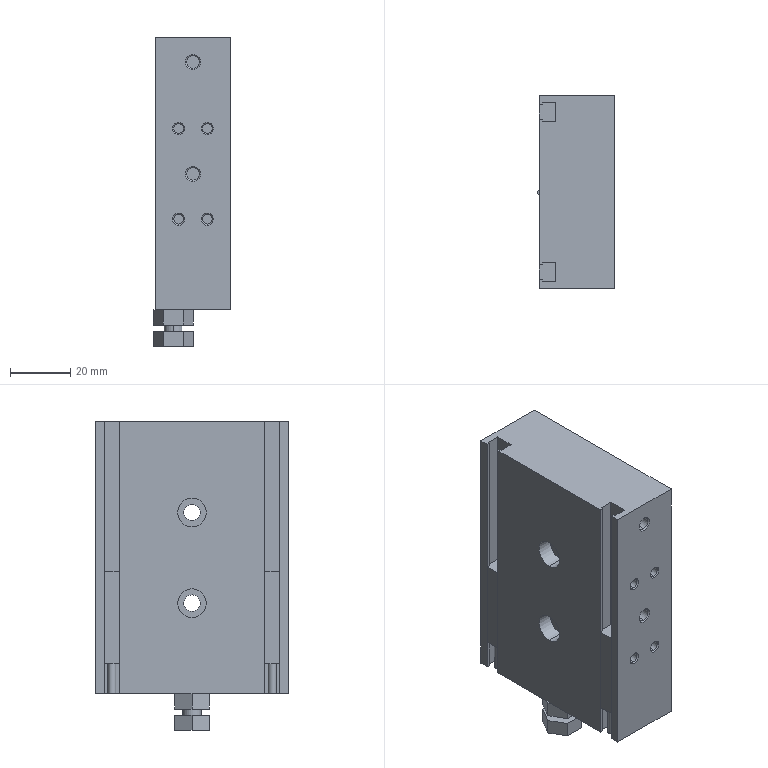Component | SolidWorks | P-SLJ-005-3_CXSM20-20-Z73-1_body CXSM20-20-Z73-1 | 1 solid | 147 faces | box 25.64 x 64 x 102 mm | volume 135415 mm3 | plane 75 | cylinder 44 | cone 28 | commonest cylinder face diameters 3.24 x16 4.13 x8 10.2 x4 2.7 x4 9.5 x4 5.5 x4 6 x4
build123d program:
from build123d import *

# Parameters (mm, degrees)
EXTRUDE1_DEPTH = 90
SKETCH2_W      = 12
SKETCH2_H      = 3
EXTRUDE2_DEPTH = 5
EXTRUDE3_DEPTH = 5
EXTRUDE4_DEPTH = 30.5
EXTRUDE5_DEPTH = 30.5
SKETCH9_R      = 1.35
EXTRUDE6_DEPTH = 10
SKETCH10_R     = 1.35
EXTRUDE7_DEPTH = 10
SKETCH23_R     = 5.1
EXTRUDE8_DEPTH = 22
SKETCH24_R     = 5.1
EXTRUDE9_DEPTH = 22


with BuildPart() as part:
    # Sketch1 → Extrude1 (new body)
    with BuildSketch(Plane.XY):
        Polygon((-32, 0), (32, 0), (32, 25), (29, 25), (29, 24), (29.65, 24), (29.65, 19.5), (23.35, 19.5), (23.35, 24), (24, 24), (24, 25), (-24, 25), (-24, 24), (-23.35, 24), (-23.35, 19.5), (-29.65, 19.5), (-29.65, 24), (-29, 24), (-29, 25), (-32, 25), align=None)
    extrude(amount=-EXTRUDE1_DEPTH)

    # Sketch2 → Revolve1 (revolve)
    with BuildSketch(Plane(origin=(0, 0, 0), x_dir=(0, 0, -1), z_dir=(1, 0, 0)), mode=Mode.PRIVATE) as revolve1_sk:
        with Locations((-6, 20.5)):
            Rectangle(SKETCH2_W, SKETCH2_H)
    revolve(revolve1_sk.sketch.rotate(Axis((0, 19, 0), (0, 0, 1)), 270), axis=Axis((0, 19, 0), (0, 0, 1)))

    # Sketch3 → Extrude2 (add)
    with BuildSketch(Plane.XY):
        Polygon((-5.75, 22.32), (-5.75, 15.68), (0, 12.36), (5.75, 15.68), (5.75, 22.32), (0, 25.64), align=None)
    extrude(amount=EXTRUDE2_DEPTH)

    # Sketch4 → Extrude3 (add)
    with BuildSketch(Plane.XY.offset(11.99)):
        Polygon((-5.75, 22.32), (-5.75, 15.68), (0, 12.36), (5.75, 15.68), (5.75, 22.32), (0, 25.64), align=None)
    extrude(amount=-EXTRUDE3_DEPTH)

    # Sketch5 → Cut-Revolve1 (revolve, cut)
    with BuildSketch(Plane(origin=(0, 0, 0), x_dir=(0, 0, -1), z_dir=(1, 0, 0)), mode=Mode.PRIVATE) as cut_revolve1_sk:
        Polygon((30, -0.5), (26.5, -0.5), (27.25, 0.25), (27.25, 19.7), (25.25, 19.7), (25.25, 25), (30, 25), align=None)
    revolve(cut_revolve1_sk.sketch.rotate(Axis((0, 25, -30), (0, -1, 0)), 180), axis=Axis((0, 25, -30), (0, -1, 0)), mode=Mode.SUBTRACT)

    # Sketch6 → Cut-Revolve2 (revolve, cut)
    with BuildSketch(Plane(origin=(0, 0, 0), x_dir=(0, 0, -1), z_dir=(1, 0, 0)), mode=Mode.PRIVATE) as cut_revolve2_sk:
        Polygon((60, -0.5), (56.5, -0.5), (57.25, 0.25), (57.25, 19.7), (55.25, 19.7), (55.25, 25), (60, 25), align=None)
    revolve(cut_revolve2_sk.sketch.rotate(Axis((0, 25, -60), (0, -1, 0)), 180), axis=Axis((0, 25, -60), (0, -1, 0)), mode=Mode.SUBTRACT)

    # Sketch7 → Extrude4 (add)
    with BuildSketch(Plane.XY.offset(-10)):
        Polygon((23.4, 19.5), (29.6, 19.5), (29.6, 24), (28.95, 24), (28.95, 25), (24.05, 25), (24.05, 24), (23.4, 24), align=None)
    extrude(amount=-EXTRUDE4_DEPTH)

    # Sketch8 → Extrude5 (add)
    with BuildSketch(Plane.XY.offset(-10)):
        Polygon((-29.6, 19.5), (-23.4, 19.5), (-23.4, 24), (-24.05, 24), (-24.05, 25), (-28.95, 25), (-28.95, 24), (-29.6, 24), align=None)
    extrude(amount=-EXTRUDE5_DEPTH)

    # Sketch9 → Extrude6 (add)
    with BuildSketch(Plane.XY.offset(-10)):
        with Locations((26.5, 22.25)):
            Circle(SKETCH9_R)
    extrude(amount=EXTRUDE6_DEPTH)

    # Sketch10 → Extrude7 (add)
    with BuildSketch(Plane.XY.offset(-10)):
        with Locations((-26.5, 22.25)):
            Circle(SKETCH10_R)
    extrude(amount=EXTRUDE7_DEPTH)

    # Sketch11 → Cut-Revolve3 (revolve, cut)
    with BuildSketch(Plane.XY.offset(-30), mode=Mode.PRIVATE) as cut_revolve3_sk:
        Polygon((26.5, 7.75), (26.5, 9.37), (31.62, 9.37), (32.5, 10.25), (32.5, 7.75), align=None)
    revolve(cut_revolve3_sk.sketch.rotate(Axis((32.5, 7.75, -30), (-1, 0, 0)), 270), axis=Axis((32.5, 7.75, -30), (-1, 0, 0)), mode=Mode.SUBTRACT)

    # Sketch12 → Cut-Revolve4 (revolve, cut)
    with BuildSketch(Plane.XY.offset(-30), mode=Mode.PRIVATE) as cut_revolve4_sk:
        Polygon((26.5, 17.25), (26.5, 18.87), (31.62, 18.87), (32.5, 19.75), (32.5, 17.25), align=None)
    revolve(cut_revolve4_sk.sketch.rotate(Axis((32.5, 17.25, -30), (-1, 0, 0)), 270), axis=Axis((32.5, 17.25, -30), (-1, 0, 0)), mode=Mode.SUBTRACT)

    # Sketch13 → Cut-Revolve5 (revolve, cut)
    with BuildSketch(Plane.XY.offset(-30), mode=Mode.PRIVATE) as cut_revolve5_sk:
        Polygon((-32.5, 7.75), (-32.5, 10.25), (-31.62, 9.37), (-26.5, 9.37), (-26.5, 7.75), align=None)
    revolve(cut_revolve5_sk.sketch.rotate(Axis((-26.5, 7.75, -30), (-1, 0, 0)), 270), axis=Axis((-26.5, 7.75, -30), (-1, 0, 0)), mode=Mode.SUBTRACT)

    # Sketch14 → Cut-Revolve6 (revolve, cut)
    with BuildSketch(Plane.XY.offset(-30), mode=Mode.PRIVATE) as cut_revolve6_sk:
        Polygon((-32.5, 17.25), (-32.5, 19.75), (-31.62, 18.87), (-26.5, 18.87), (-26.5, 17.25), align=None)
    revolve(cut_revolve6_sk.sketch.rotate(Axis((-26.5, 17.25, -30), (-1, 0, 0)), 270), axis=Axis((-26.5, 17.25, -30), (-1, 0, 0)), mode=Mode.SUBTRACT)

    # Sketch15 → Cut-Revolve7 (revolve, cut)
    with BuildSketch(Plane.XY.offset(-60), mode=Mode.PRIVATE) as cut_revolve7_sk:
        Polygon((26.5, 7.75), (26.5, 9.37), (31.62, 9.37), (32.5, 10.25), (32.5, 7.75), align=None)
    revolve(cut_revolve7_sk.sketch.rotate(Axis((32.5, 7.75, -60), (-1, 0, 0)), 270), axis=Axis((32.5, 7.75, -60), (-1, 0, 0)), mode=Mode.SUBTRACT)

    # Sketch16 → Cut-Revolve8 (revolve, cut)
    with BuildSketch(Plane.XY.offset(-60), mode=Mode.PRIVATE) as cut_revolve8_sk:
        Polygon((26.5, 17.25), (26.5, 18.87), (31.62, 18.87), (32.5, 19.75), (32.5, 17.25), align=None)
    revolve(cut_revolve8_sk.sketch.rotate(Axis((32.5, 17.25, -60), (-1, 0, 0)), 270), axis=Axis((32.5, 17.25, -60), (-1, 0, 0)), mode=Mode.SUBTRACT)

    # Sketch17 → Cut-Revolve9 (revolve, cut)
    with BuildSketch(Plane.XY.offset(-60), mode=Mode.PRIVATE) as cut_revolve9_sk:
        Polygon((-32.5, 7.75), (-32.5, 10.25), (-31.62, 9.37), (-26.5, 9.37), (-26.5, 7.75), align=None)
    revolve(cut_revolve9_sk.sketch.rotate(Axis((-26.5, 7.75, -60), (-1, 0, 0)), 270), axis=Axis((-26.5, 7.75, -60), (-1, 0, 0)), mode=Mode.SUBTRACT)

    # Sketch18 → Cut-Revolve10 (revolve, cut)
    with BuildSketch(Plane.XY.offset(-60), mode=Mode.PRIVATE) as cut_revolve10_sk:
        Polygon((-32.5, 17.25), (-32.5, 19.75), (-31.62, 18.87), (-26.5, 18.87), (-26.5, 17.25), align=None)
    revolve(cut_revolve10_sk.sketch.rotate(Axis((-26.5, 17.25, -60), (-1, 0, 0)), 270), axis=Axis((-26.5, 17.25, -60), (-1, 0, 0)), mode=Mode.SUBTRACT)

    # Sketch19 → Cut-Revolve11 (revolve, cut)
    with BuildSketch(Plane(origin=(0, 12.5, 0), x_dir=(1, 0, 0), z_dir=(0, 1, 0)), mode=Mode.PRIVATE) as cut_revolve11_sk:
        Polygon((27.5, 45), (27.5, 47.065), (31.565, 47.065), (32.5, 48), (32.5, 45), align=None)
    revolve(cut_revolve11_sk.sketch.rotate(Axis((32.5, 12.5, -45), (-1, 0, 0)), 180), axis=Axis((32.5, 12.5, -45), (-1, 0, 0)), mode=Mode.SUBTRACT)

    # Sketch20 → Cut-Revolve12 (revolve, cut)
    with BuildSketch(Plane(origin=(0, 12.5, 0), x_dir=(1, 0, 0), z_dir=(0, 1, 0)), mode=Mode.PRIVATE) as cut_revolve12_sk:
        Polygon((-32.5, 45), (-32.5, 48), (-31.565, 47.065), (-27.5, 47.065), (-27.5, 45), align=None)
    revolve(cut_revolve12_sk.sketch.rotate(Axis((-27.5, 12.5, -45), (-1, 0, 0)), 180), axis=Axis((-27.5, 12.5, -45), (-1, 0, 0)), mode=Mode.SUBTRACT)

    # Sketch21 → Cut-Revolve13 (revolve, cut)
    with BuildSketch(Plane(origin=(0, 12.5, 0), x_dir=(1, 0, 0), z_dir=(0, 1, 0)), mode=Mode.PRIVATE) as cut_revolve13_sk:
        Polygon((27.5, 82), (27.5, 84.065), (31.565, 84.065), (32.5, 85), (32.5, 82), align=None)
    revolve(cut_revolve13_sk.sketch.rotate(Axis((32.5, 12.5, -82), (-1, 0, 0)), 180), axis=Axis((32.5, 12.5, -82), (-1, 0, 0)), mode=Mode.SUBTRACT)

    # Sketch22 → Cut-Revolve14 (revolve, cut)
    with BuildSketch(Plane(origin=(0, 12.5, 0), x_dir=(1, 0, 0), z_dir=(0, 1, 0)), mode=Mode.PRIVATE) as cut_revolve14_sk:
        Polygon((-32.5, 82), (-32.5, 85), (-31.565, 84.065), (-27.5, 84.065), (-27.5, 82), align=None)
    revolve(cut_revolve14_sk.sketch.rotate(Axis((-27.5, 12.5, -82), (-1, 0, 0)), 180), axis=Axis((-27.5, 12.5, -82), (-1, 0, 0)), mode=Mode.SUBTRACT)

    # Sketch23 → Extrude8 (cut)
    with BuildSketch(Plane.XY):
        with Locations((14, 12.5)):
            Circle(SKETCH23_R)
    extrude(amount=-EXTRUDE8_DEPTH, mode=Mode.SUBTRACT)

    # Sketch24 → Extrude9 (cut)
    with BuildSketch(Plane.XY):
        with Locations((-14, 12.5)):
            Circle(SKETCH24_R)
    extrude(amount=-EXTRUDE9_DEPTH, mode=Mode.SUBTRACT)


solid = part.part

# Placed as in the assembly
solid = solid.moved(Location((-49.5, 15.5, 1287.634), (180, 0, 90)))